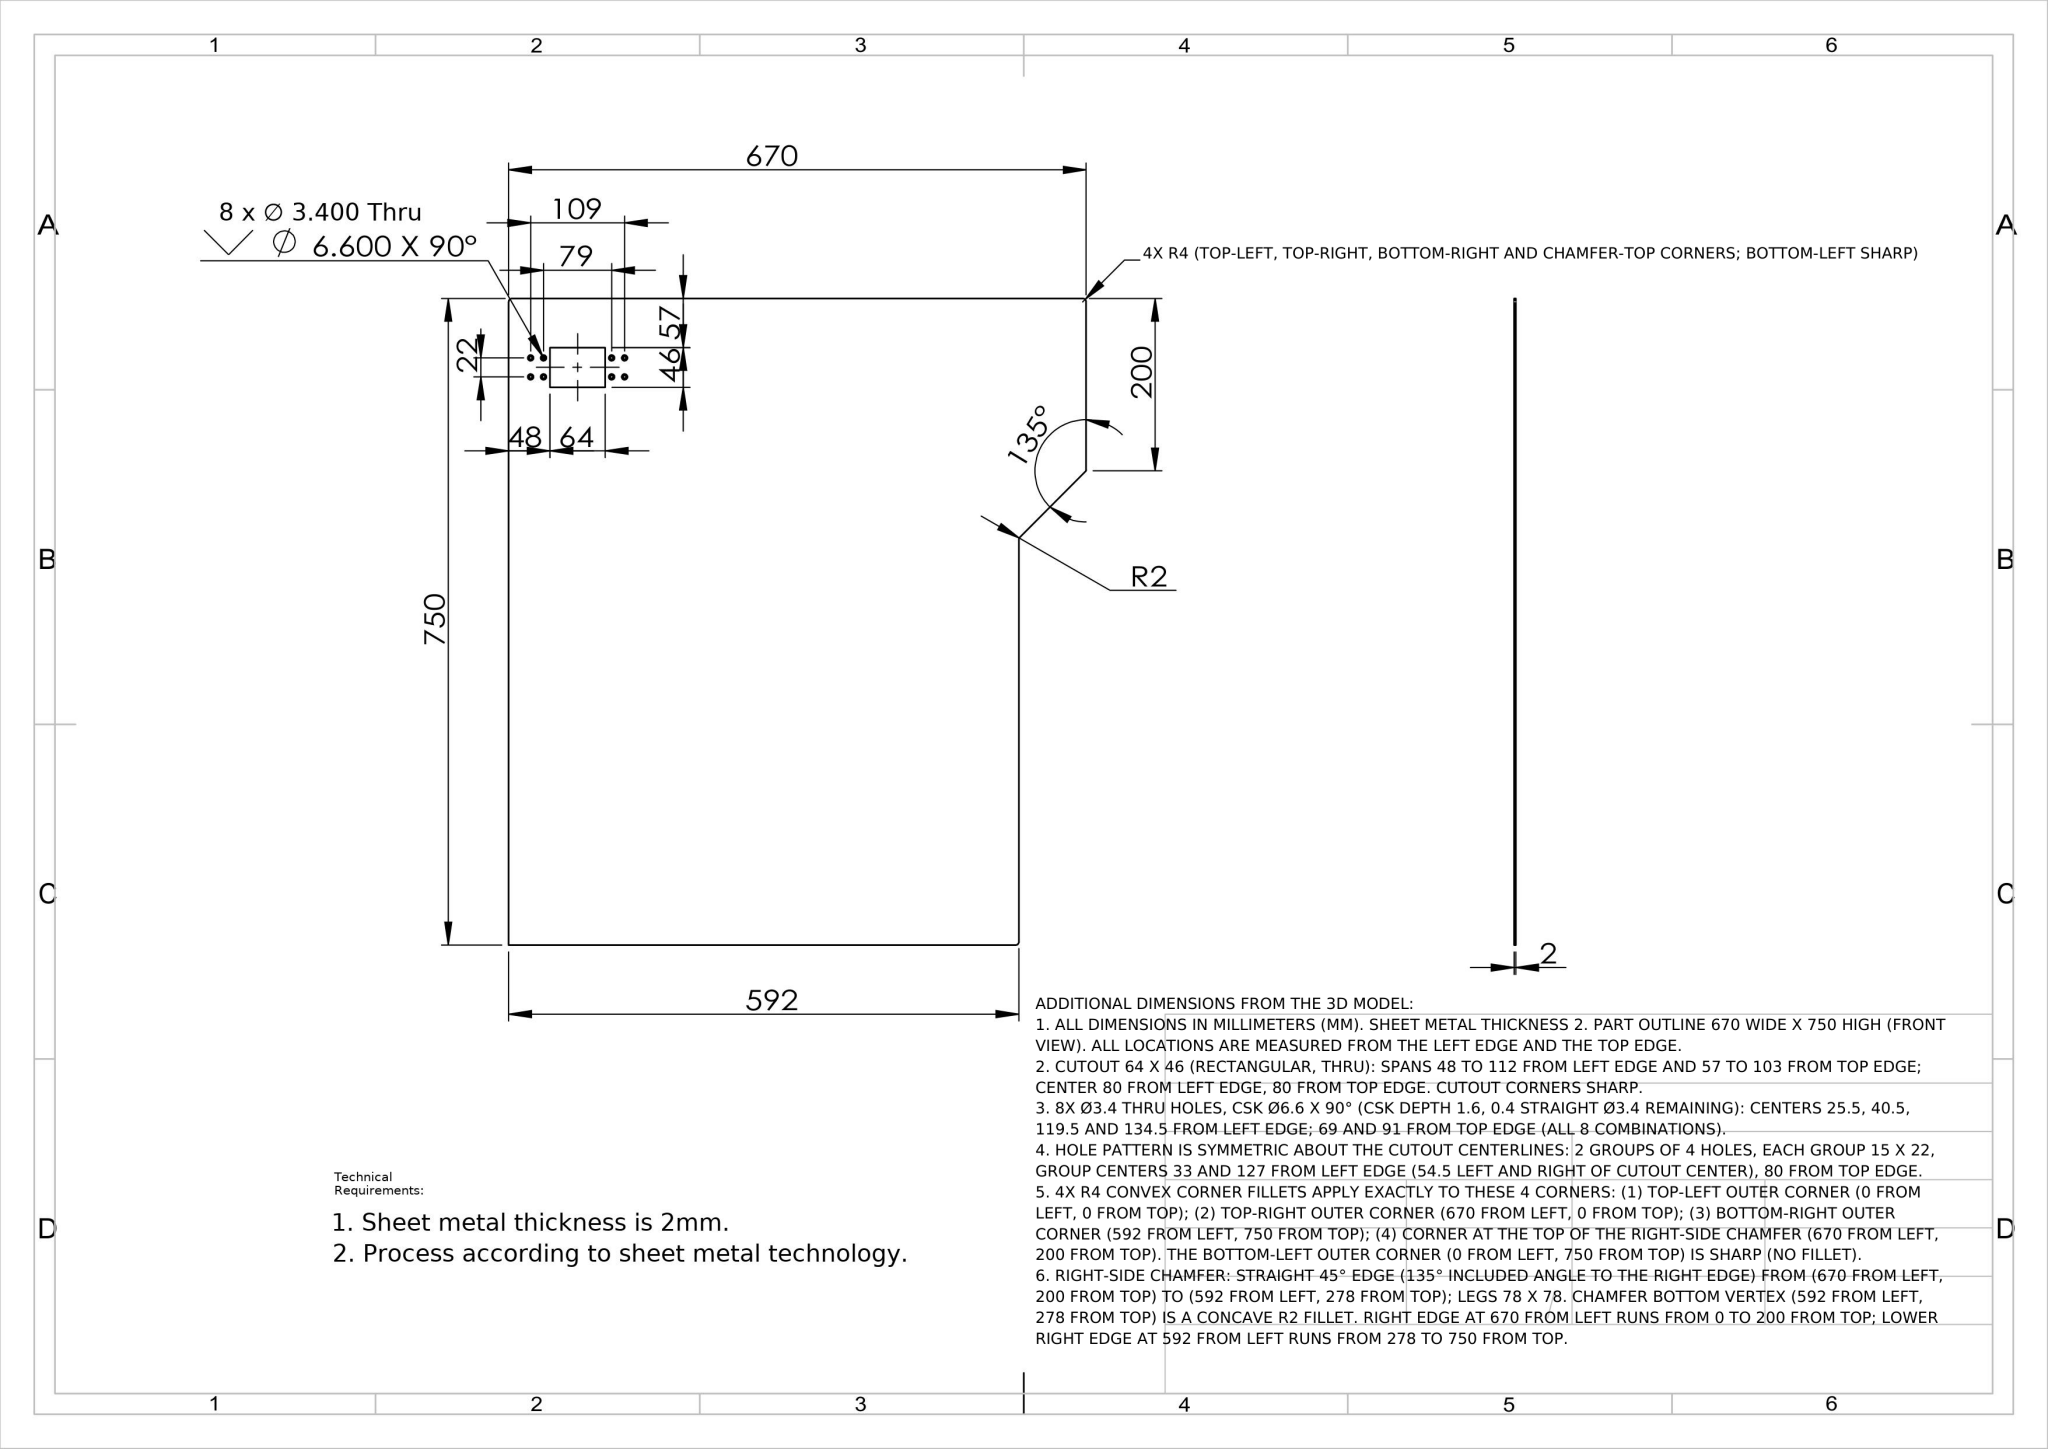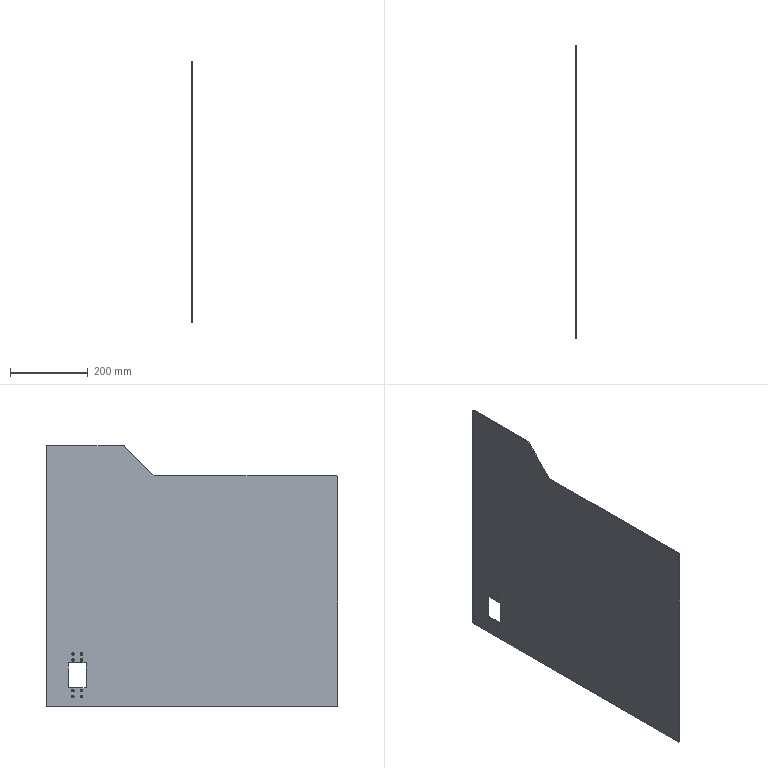Part | NX | mm | 1 solid | 49 faces | box 2 x 750 x 670 mm | volume 919086 mm3 | cylinder 21 | cone 16 | plane 12 | commonest cylinder face diameters 3.4 x16 8 x4 4 x1